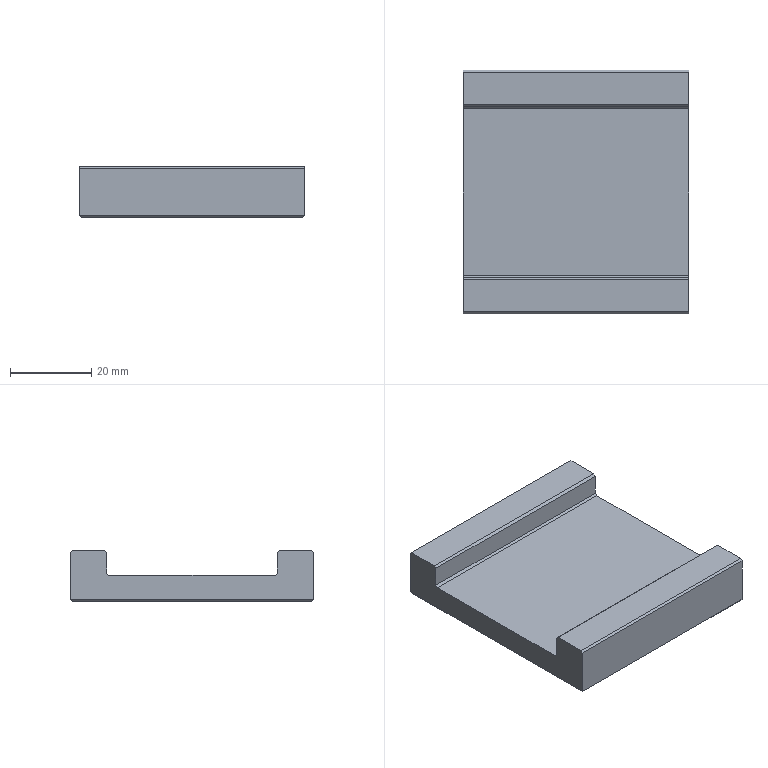Component | SolidWorks | SRS15WM-Slider-2-1 | 1 solid | 36 faces | box 55.5 x 60 x 12.6 mm | volume 27480 mm3 | plane 20 | cylinder 8 | cone 8 | commonest cylinder face diameters 3.3 x8
build123d program:
from build123d import *

# Parameters (mm, degrees)
BOSS_EXTRUDE1_DEPTH   = 55.5
CHAMFER1_SIZE         = 0.5
M4_TAPPED_HOLE1_D     = 3.3
M4_TAPPED_HOLE1_DEPTH = 6
M4_TAPPED_HOLE1_TIP   = 0.9914


with BuildPart() as part:
    # Sketch1 → Boss-Extrude1 (new body)
    with BuildSketch(Plane.XY):
        Polygon((9, 0), (9, 6.1), (51, 6.1), (51, 0), (60, 0), (60, 12.6), (0, 12.6), (0, 0), align=None)
    extrude(amount=BOSS_EXTRUDE1_DEPTH)

    # Chamfer1
    chamfer1_edges = [part.edges().sort_by_distance(p)[0] for p in [
        (0, 12.6, 27.75),
        (60, 12.6, 27.75),
        (60, 0, 27.75),
        (51, 0, 27.75),
        (51, 6.1, 27.75),
        (9, 6.1, 27.75),
        (9, 0, 27.75),
        (0, 0, 27.75),
        (30, 12.6, 55.5),
        (30, 12.6, 0),
    ]]
    chamfer(chamfer1_edges, length=CHAMFER1_SIZE)

    # M4 Tapped Hole1
    with Locations(Plane(origin=(0, 12.6, 0), x_dir=(1, 0, 0), z_dir=(0, 1, 0))):
        with Locations((7.5, -17.75), (52.5, -17.75), (52.5, -37.75), (7.5, -37.75)):
            Hole(M4_TAPPED_HOLE1_D / 2, depth=M4_TAPPED_HOLE1_DEPTH)
            with Locations((0, 0, -(M4_TAPPED_HOLE1_DEPTH + M4_TAPPED_HOLE1_TIP / 2))):  # 118° drill point
                Cone(0, M4_TAPPED_HOLE1_D / 2, M4_TAPPED_HOLE1_TIP, mode=Mode.SUBTRACT)


solid = part.part

# Placed as in the assembly
solid = solid.moved(Location((-73.445, 49.945, 33.151), (-90, 90, 0)))
STEP:
#1=COLOUR_RGB('',0.7922,0.8196,0.9333);
#2=FILL_AREA_STYLE_COLOUR('',#1);
#3=FILL_AREA_STYLE('',(#2));
#4=SURFACE_STYLE_FILL_AREA(#3);
#5=SURFACE_SIDE_STYLE('',(#4));
#6=SURFACE_STYLE_USAGE(.BOTH.,#5);
#7=PRESENTATION_STYLE_ASSIGNMENT((#6));
#8=CARTESIAN_POINT('',(-1.34,-0.1006,1.045));
#9=VERTEX_POINT('',#8);
#10=CARTESIAN_POINT('',(-1.47,-0.1006,1.045));
#11=VERTEX_POINT('',#10);
#12=CARTESIAN_POINT('',(-1.405,-0.1006,1.045));
#13=DIRECTION('',(-0.,0.,-1.));
#14=DIRECTION('',(-1.,0.,0.));
#15=AXIS2_PLACEMENT_3D('',#12,#13,#14);
#16=CIRCLE('',#15,0.06496);
#17=EDGE_CURVE('',#9,#11,#16,.T.);
#18=ORIENTED_EDGE('',*,*,#17,.F.);
#19=CARTESIAN_POINT('',(-1.34,-0.1006,0.8091));
#20=VERTEX_POINT('',#19);
#21=CARTESIAN_POINT('',(-1.34,-0.1006,0.8091));
#22=DIRECTION('',(-0.,0.,-1.));
#23=VECTOR('',#22,39.37);
#24=LINE('',#21,#23);
#25=EDGE_CURVE('',#9,#20,#24,.T.);
#26=ORIENTED_EDGE('',*,*,#25,.T.);
#27=CARTESIAN_POINT('',(-1.47,-0.1006,0.8091));
#28=VERTEX_POINT('',#27);
#29=CARTESIAN_POINT('',(-1.405,-0.1006,0.8091));
#30=DIRECTION('',(-0.,0.,-1.));
#31=DIRECTION('',(-1.,0.,0.));
#32=AXIS2_PLACEMENT_3D('',#29,#30,#31);
#33=CIRCLE('',#32,0.06496);
#34=EDGE_CURVE('',#20,#28,#33,.T.);
#35=ORIENTED_EDGE('',*,*,#34,.T.);
#36=CARTESIAN_POINT('',(-1.47,-0.1006,0.8091));
#37=DIRECTION('',(-0.,0.,-1.));
#38=VECTOR('',#37,39.37);
#39=LINE('',#36,#38);
#40=EDGE_CURVE('',#11,#28,#39,.T.);
#41=ORIENTED_EDGE('',*,*,#40,.F.);
#42=EDGE_LOOP('',(#18,#26,#35,#41));
#43=FACE_OUTER_BOUND('',#42,.T.);
#44=CARTESIAN_POINT('',(-1.405,-0.1006,0.8091));
#45=DIRECTION('',(-0.,0.,-1.));
#46=DIRECTION('',(-1.,0.,0.));
#47=AXIS2_PLACEMENT_3D('',#44,#45,#46);
#48=CYLINDRICAL_SURFACE('',#47,0.06496);
#49=ADVANCED_FACE('',(#43),#48,.F.);
#50=CARTESIAN_POINT('',(-1.405,-0.1006,1.084));
#51=VERTEX_POINT('',#50);
#52=CARTESIAN_POINT('',(-1.47,-0.1006,1.045));
#53=DIRECTION('',(-0.8572,0.,-0.515));
#54=VECTOR('',#53,39.37);
#55=LINE('',#52,#54);
#56=EDGE_CURVE('',#51,#11,#55,.T.);
#57=ORIENTED_EDGE('',*,*,#56,.F.);
#58=CARTESIAN_POINT('',(-1.34,-0.1006,1.045));
#59=DIRECTION('',(0.8572,-0.,-0.515));
#60=VECTOR('',#59,39.37);
#61=LINE('',#58,#60);
#62=EDGE_CURVE('',#51,#9,#61,.T.);
#63=ORIENTED_EDGE('',*,*,#62,.T.);
#64=ORIENTED_EDGE('',*,*,#17,.T.);
#65=EDGE_LOOP('',(#57,#63,#64));
#66=FACE_OUTER_BOUND('',#65,.T.);
#67=CARTESIAN_POINT('',(-1.405,-0.1006,1.045));
#68=DIRECTION('',(-0.,0.,-1.));
#69=DIRECTION('',(-1.,0.,0.));
#70=AXIS2_PLACEMENT_3D('',#67,#68,#69);
#71=CONICAL_SURFACE('',#70,0.06496,1.03);
#72=ADVANCED_FACE('',(#66),#71,.F.);
#73=CARTESIAN_POINT('',(-1.34,1.671,1.045));
#74=VERTEX_POINT('',#73);
#75=CARTESIAN_POINT('',(-1.47,1.671,1.045));
#76=VERTEX_POINT('',#75);
#77=CARTESIAN_POINT('',(-1.405,1.671,1.045));
#78=DIRECTION('',(-0.,0.,-1.));
#79=DIRECTION('',(-1.,0.,0.));
#80=AXIS2_PLACEMENT_3D('',#77,#78,#79);
#81=CIRCLE('',#80,0.06496);
#82=EDGE_CURVE('',#74,#76,#81,.T.);
#83=ORIENTED_EDGE('',*,*,#82,.F.);
#84=CARTESIAN_POINT('',(-1.34,1.671,0.8091));
#85=VERTEX_POINT('',#84);
#86=CARTESIAN_POINT('',(-1.34,1.671,0.8091));
#87=DIRECTION('',(-0.,0.,-1.));
#88=VECTOR('',#87,39.37);
#89=LINE('',#86,#88);
#90=EDGE_CURVE('',#74,#85,#89,.T.);
#91=ORIENTED_EDGE('',*,*,#90,.T.);
#92=CARTESIAN_POINT('',(-1.47,1.671,0.8091));
#93=VERTEX_POINT('',#92);
#94=CARTESIAN_POINT('',(-1.405,1.671,0.8091));
#95=DIRECTION('',(-0.,0.,-1.));
#96=DIRECTION('',(-1.,0.,0.));
#97=AXIS2_PLACEMENT_3D('',#94,#95,#96);
#98=CIRCLE('',#97,0.06496);
#99=EDGE_CURVE('',#85,#93,#98,.T.);
#100=ORIENTED_EDGE('',*,*,#99,.T.);
#101=CARTESIAN_POINT('',(-1.47,1.671,0.8091));
#102=DIRECTION('',(-0.,0.,-1.));
#103=VECTOR('',#102,39.37);
#104=LINE('',#101,#103);
#105=EDGE_CURVE('',#76,#93,#104,.T.);
#106=ORIENTED_EDGE('',*,*,#105,.F.);
#107=EDGE_LOOP('',(#83,#91,#100,#106));
#108=FACE_OUTER_BOUND('',#107,.T.);
#109=CARTESIAN_POINT('',(-1.405,1.671,0.8091));
#110=DIRECTION('',(-0.,0.,-1.));
#111=DIRECTION('',(-1.,0.,0.));
#112=AXIS2_PLACEMENT_3D('',#109,#110,#111);
#113=CYLINDRICAL_SURFACE('',#112,0.06496);
#114=ADVANCED_FACE('',(#108),#113,.F.);
#115=CARTESIAN_POINT('',(-1.405,1.671,1.084));
#116=VERTEX_POINT('',#115);
#117=CARTESIAN_POINT('',(-1.47,1.671,1.045));
#118=DIRECTION('',(-0.8572,0.,-0.515));
#119=VECTOR('',#118,39.37);
#120=LINE('',#117,#119);
#121=EDGE_CURVE('',#116,#76,#120,.T.);
#122=ORIENTED_EDGE('',*,*,#121,.F.);
#123=CARTESIAN_POINT('',(-1.34,1.671,1.045));
#124=DIRECTION('',(0.8572,-0.,-0.515));
#125=VECTOR('',#124,39.37);
#126=LINE('',#123,#125);
#127=EDGE_CURVE('',#116,#74,#126,.T.);
#128=ORIENTED_EDGE('',*,*,#127,.T.);
#129=ORIENTED_EDGE('',*,*,#82,.T.);
#130=EDGE_LOOP('',(#122,#128,#129));
#131=FACE_OUTER_BOUND('',#130,.T.);
#132=CARTESIAN_POINT('',(-1.405,1.671,1.045));
#133=DIRECTION('',(-0.,0.,-1.));
#134=DIRECTION('',(-1.,0.,0.));
#135=AXIS2_PLACEMENT_3D('',#132,#133,#134);
#136=CONICAL_SURFACE('',#135,0.06496,1.03);
#137=ADVANCED_FACE('',(#131),#136,.F.);
#138=CARTESIAN_POINT('',(-2.128,1.671,1.045));
#139=VERTEX_POINT('',#138);
#140=CARTESIAN_POINT('',(-2.258,1.671,1.045));
#141=VERTEX_POINT('',#140);
#142=CARTESIAN_POINT('',(-2.193,1.671,1.045));
#143=DIRECTION('',(-0.,0.,-1.));
#144=DIRECTION('',(-1.,0.,0.));
#145=AXIS2_PLACEMENT_3D('',#142,#143,#144);
#146=CIRCLE('',#145,0.06496);
#147=EDGE_CURVE('',#139,#141,#146,.T.);
#148=ORIENTED_EDGE('',*,*,#147,.F.);
#149=CARTESIAN_POINT('',(-2.128,1.671,0.8091));
#150=VERTEX_POINT('',#149);
#151=CARTESIAN_POINT('',(-2.128,1.671,0.8091));
#152=DIRECTION('',(-0.,0.,-1.));
#153=VECTOR('',#152,39.37);
#154=LINE('',#151,#153);
#155=EDGE_CURVE('',#139,#150,#154,.T.);
#156=ORIENTED_EDGE('',*,*,#155,.T.);
#157=CARTESIAN_POINT('',(-2.258,1.671,0.8091));
#158=VERTEX_POINT('',#157);
#159=CARTESIAN_POINT('',(-2.193,1.671,0.8091));
#160=DIRECTION('',(-0.,0.,-1.));
#161=DIRECTION('',(-1.,0.,0.));
#162=AXIS2_PLACEMENT_3D('',#159,#160,#161);
#163=CIRCLE('',#162,0.06496);
#164=EDGE_CURVE('',#150,#158,#163,.T.);
#165=ORIENTED_EDGE('',*,*,#164,.T.);
#166=CARTESIAN_POINT('',(-2.258,1.671,0.8091));
#167=DIRECTION('',(-0.,0.,-1.));
#168=VECTOR('',#167,39.37);
#169=LINE('',#166,#168);
#170=EDGE_CURVE('',#141,#158,#169,.T.);
#171=ORIENTED_EDGE('',*,*,#170,.F.);
#172=EDGE_LOOP('',(#148,#156,#165,#171));
#173=FACE_OUTER_BOUND('',#172,.T.);
#174=CARTESIAN_POINT('',(-2.193,1.671,0.8091));
#175=DIRECTION('',(-0.,0.,-1.));
#176=DIRECTION('',(-1.,0.,0.));
#177=AXIS2_PLACEMENT_3D('',#174,#175,#176);
#178=CYLINDRICAL_SURFACE('',#177,0.06496);
#179=ADVANCED_FACE('',(#173),#178,.F.);
#180=CARTESIAN_POINT('',(-2.193,1.671,1.084));
#181=VERTEX_POINT('',#180);
#182=CARTESIAN_POINT('',(-2.258,1.671,1.045));
#183=DIRECTION('',(-0.8572,0.,-0.515));
#184=VECTOR('',#183,39.37);
#185=LINE('',#182,#184);
#186=EDGE_CURVE('',#181,#141,#185,.T.);
#187=ORIENTED_EDGE('',*,*,#186,.F.);
#188=CARTESIAN_POINT('',(-2.128,1.671,1.045));
#189=DIRECTION('',(0.8572,-0.,-0.515));
#190=VECTOR('',#189,39.37);
#191=LINE('',#188,#190);
#192=EDGE_CURVE('',#181,#139,#191,.T.);
#193=ORIENTED_EDGE('',*,*,#192,.T.);
#194=ORIENTED_EDGE('',*,*,#147,.T.);
#195=EDGE_LOOP('',(#187,#193,#194));
#196=FACE_OUTER_BOUND('',#195,.T.);
#197=CARTESIAN_POINT('',(-2.193,1.671,1.045));
#198=DIRECTION('',(-0.,0.,-1.));
#199=DIRECTION('',(-1.,0.,0.));
#200=AXIS2_PLACEMENT_3D('',#197,#198,#199);
#201=CONICAL_SURFACE('',#200,0.06496,1.03);
#202=ADVANCED_FACE('',(#196),#201,.F.);
#203=CARTESIAN_POINT('',(-2.128,-0.1006,1.045));
#204=VERTEX_POINT('',#203);
#205=CARTESIAN_POINT('',(-2.258,-0.1006,1.045));
#206=VERTEX_POINT('',#205);
#207=CARTESIAN_POINT('',(-2.193,-0.1006,1.045));
#208=DIRECTION('',(-0.,0.,-1.));
#209=DIRECTION('',(-1.,0.,0.));
#210=AXIS2_PLACEMENT_3D('',#207,#208,#209);
#211=CIRCLE('',#210,0.06496);
#212=EDGE_CURVE('',#204,#206,#211,.T.);
#213=ORIENTED_EDGE('',*,*,#212,.F.);
#214=CARTESIAN_POINT('',(-2.128,-0.1006,0.8091));
#215=VERTEX_POINT('',#214);
#216=CARTESIAN_POINT('',(-2.128,-0.1006,0.8091));
#217=DIRECTION('',(-0.,0.,-1.));
#218=VECTOR('',#217,39.37);
#219=LINE('',#216,#218);
#220=EDGE_CURVE('',#204,#215,#219,.T.);
#221=ORIENTED_EDGE('',*,*,#220,.T.);
#222=CARTESIAN_POINT('',(-2.258,-0.1006,0.8091));
#223=VERTEX_POINT('',#222);
#224=CARTESIAN_POINT('',(-2.193,-0.1006,0.8091));
#225=DIRECTION('',(-0.,0.,-1.));
#226=DIRECTION('',(-1.,0.,0.));
#227=AXIS2_PLACEMENT_3D('',#224,#225,#226);
#228=CIRCLE('',#227,0.06496);
#229=EDGE_CURVE('',#215,#223,#228,.T.);
#230=ORIENTED_EDGE('',*,*,#229,.T.);
#231=CARTESIAN_POINT('',(-2.258,-0.1006,0.8091));
#232=DIRECTION('',(-0.,0.,-1.));
#233=VECTOR('',#232,39.37);
#234=LINE('',#231,#233);
#235=EDGE_CURVE('',#206,#223,#234,.T.);
#236=ORIENTED_EDGE('',*,*,#235,.F.);
#237=EDGE_LOOP('',(#213,#221,#230,#236));
#238=FACE_OUTER_BOUND('',#237,.T.);
#239=CARTESIAN_POINT('',(-2.193,-0.1006,0.8091));
#240=DIRECTION('',(-0.,0.,-1.));
#241=DIRECTION('',(-1.,0.,0.));
#242=AXIS2_PLACEMENT_3D('',#239,#240,#241);
#243=CYLINDRICAL_SURFACE('',#242,0.06496);
#244=ADVANCED_FACE('',(#238),#243,.F.);
#245=CARTESIAN_POINT('',(-2.193,-0.1006,1.084));
#246=VERTEX_POINT('',#245);
#247=CARTESIAN_POINT('',(-2.258,-0.1006,1.045));
#248=DIRECTION('',(-0.8572,0.,-0.515));
#249=VECTOR('',#248,39.37);
#250=LINE('',#247,#249);
#251=EDGE_CURVE('',#246,#206,#250,.T.);
#252=ORIENTED_EDGE('',*,*,#251,.F.);
#253=CARTESIAN_POINT('',(-2.128,-0.1006,1.045));
#254=DIRECTION('',(0.8572,-0.,-0.515));
#255=VECTOR('',#254,39.37);
#256=LINE('',#253,#255);
#257=EDGE_CURVE('',#246,#204,#256,.T.);
#258=ORIENTED_EDGE('',*,*,#257,.T.);
#259=ORIENTED_EDGE('',*,*,#212,.T.);
#260=EDGE_LOOP('',(#252,#258,#259));
#261=FACE_OUTER_BOUND('',#260,.T.);
#262=CARTESIAN_POINT('',(-2.193,-0.1006,1.045));
#263=DIRECTION('',(-0.,0.,-1.));
#264=DIRECTION('',(-1.,0.,0.));
#265=AXIS2_PLACEMENT_3D('',#262,#263,#264);
#266=CONICAL_SURFACE('',#265,0.06496,1.03);
#267=ADVANCED_FACE('',(#261),#266,.F.);
#268=CARTESIAN_POINT('',(-2.892,-0.3959,0.8288));
#269=VERTEX_POINT('',#268);
#270=CARTESIAN_POINT('',(-2.892,-0.3959,1.285));
#271=VERTEX_POINT('',#270);
#272=CARTESIAN_POINT('',(-2.892,-0.3959,1.305));
#273=DIRECTION('',(0.,-0.,1.));
#274=VECTOR('',#273,39.37);
#275=LINE('',#272,#274);
#276=EDGE_CURVE('',#269,#271,#275,.T.);
#277=ORIENTED_EDGE('',*,*,#276,.F.);
#278=CARTESIAN_POINT('',(-0.7065,-0.3959,0.8288));
#279=VERTEX_POINT('',#278);
#280=CARTESIAN_POINT('',(-2.892,-0.3959,0.8288));
#281=DIRECTION('',(1.,-0.,-0.));
#282=VECTOR('',#281,39.37);
#283=LINE('',#280,#282);
#284=EDGE_CURVE('',#269,#279,#283,.T.);
#285=ORIENTED_EDGE('',*,*,#284,.T.);
#286=CARTESIAN_POINT('',(-0.7065,-0.3959,1.285));
#287=VERTEX_POINT('',#286);
#288=CARTESIAN_POINT('',(-0.7065,-0.3959,1.305));
#289=DIRECTION('',(0.,-0.,1.));
#290=VECTOR('',#289,39.37);
#291=LINE('',#288,#290);
#292=EDGE_CURVE('',#279,#287,#291,.T.);
#293=ORIENTED_EDGE('',*,*,#292,.T.);
#294=CARTESIAN_POINT('',(-2.892,-0.3959,1.285));
#295=DIRECTION('',(-1.,0.,0.));
#296=VECTOR('',#295,39.37);
#297=LINE('',#294,#296);
#298=EDGE_CURVE('',#287,#271,#297,.T.);
#299=ORIENTED_EDGE('',*,*,#298,.T.);
#300=EDGE_LOOP('',(#277,#285,#293,#299));
#301=FACE_OUTER_BOUND('',#300,.T.);
#302=CARTESIAN_POINT('',(-2.892,-0.3959,1.305));
#303=DIRECTION('',(0.,1.,0.));
#304=DIRECTION('',(1.,-0.,-0.));
#305=AXIS2_PLACEMENT_3D('',#302,#303,#304);
#306=PLANE('',#305);
#307=ADVANCED_FACE('',(#301),#306,.F.);
#308=CARTESIAN_POINT('',(-0.7065,-0.3762,1.305));
#309=VERTEX_POINT('',#308);
#310=CARTESIAN_POINT('',(-0.7065,-0.0612,1.305));
#311=VERTEX_POINT('',#310);
#312=CARTESIAN_POINT('',(-0.7065,-0.3959,1.305));
#313=DIRECTION('',(0.,1.,0.));
#314=VECTOR('',#313,39.37);
#315=LINE('',#312,#314);
#316=EDGE_CURVE('',#309,#311,#315,.T.);
#317=ORIENTED_EDGE('',*,*,#316,.T.);
#318=CARTESIAN_POINT('',(-2.892,-0.0612,1.305));
#319=VERTEX_POINT('',#318);
#320=CARTESIAN_POINT('',(-2.892,-0.0612,1.305));
#321=DIRECTION('',(-1.,0.,0.));
#322=VECTOR('',#321,39.37);
#323=LINE('',#320,#322);
#324=EDGE_CURVE('',#311,#319,#323,.T.);
#325=ORIENTED_EDGE('',*,*,#324,.T.);
#326=CARTESIAN_POINT('',(-2.892,-0.3762,1.305));
#327=VERTEX_POINT('',#326);
#328=CARTESIAN_POINT('',(-2.892,-0.3959,1.305));
#329=DIRECTION('',(0.,1.,0.));
#330=VECTOR('',#329,39.37);
#331=LINE('',#328,#330);
#332=EDGE_CURVE('',#327,#319,#331,.T.);
#333=ORIENTED_EDGE('',*,*,#332,.F.);
#334=CARTESIAN_POINT('',(-2.892,-0.3762,1.305));
#335=DIRECTION('',(1.,-0.,-0.));
#336=VECTOR('',#335,39.37);
#337=LINE('',#334,#336);
#338=EDGE_CURVE('',#327,#309,#337,.T.);
#339=ORIENTED_EDGE('',*,*,#338,.T.);
#340=EDGE_LOOP('',(#317,#325,#333,#339));
#341=FACE_OUTER_BOUND('',#340,.T.);
#342=CARTESIAN_POINT('',(-2.892,-0.3959,1.305));
#343=DIRECTION('',(-0.,0.,-1.));
#344=DIRECTION('',(-1.,0.,0.));
#345=AXIS2_PLACEMENT_3D('',#342,#343,#344);
#346=PLANE('',#345);
#347=ADVANCED_FACE('',(#341),#346,.F.);
#348=CARTESIAN_POINT('',(-0.7065,-0.04152,1.285));
#349=VERTEX_POINT('',#348);
#350=CARTESIAN_POINT('',(-0.7065,-0.04152,1.085));
#351=VERTEX_POINT('',#350);
#352=CARTESIAN_POINT('',(-0.7065,-0.04152,1.305));
#353=DIRECTION('',(-0.,0.,-1.));
#354=VECTOR('',#353,39.37);
#355=LINE('',#352,#354);
#356=EDGE_CURVE('',#349,#351,#355,.T.);
#357=ORIENTED_EDGE('',*,*,#356,.T.);
#358=CARTESIAN_POINT('',(-2.892,-0.04152,1.085));
#359=VERTEX_POINT('',#358);
#360=CARTESIAN_POINT('',(-2.892,-0.04152,1.085));
#361=DIRECTION('',(-1.,0.,0.));
#362=VECTOR('',#361,39.37);
#363=LINE('',#360,#362);
#364=EDGE_CURVE('',#351,#359,#363,.T.);
#365=ORIENTED_EDGE('',*,*,#364,.T.);
#366=CARTESIAN_POINT('',(-2.892,-0.04152,1.285));
#367=VERTEX_POINT('',#366);
#368=CARTESIAN_POINT('',(-2.892,-0.04152,1.305));
#369=DIRECTION('',(-0.,0.,-1.));
#370=VECTOR('',#369,39.37);
#371=LINE('',#368,#370);
#372=EDGE_CURVE('',#367,#359,#371,.T.);
#373=ORIENTED_EDGE('',*,*,#372,.F.);
#374=CARTESIAN_POINT('',(-2.892,-0.04152,1.285));
#375=DIRECTION('',(1.,-0.,-0.));
#376=VECTOR('',#375,39.37);
#377=LINE('',#374,#376);
#378=EDGE_CURVE('',#367,#349,#377,.T.);
#379=ORIENTED_EDGE('',*,*,#378,.T.);
#380=EDGE_LOOP('',(#357,#365,#373,#379));
#381=FACE_OUTER_BOUND('',#380,.T.);
#382=CARTESIAN_POINT('',(-2.892,-0.04152,1.305));
#383=DIRECTION('',(-0.,-1.,-0.));
#384=DIRECTION('',(-1.,0.,0.));
#385=AXIS2_PLACEMENT_3D('',#382,#383,#384);
#386=PLANE('',#385);
#387=ADVANCED_FACE('',(#381),#386,.F.);
#388=CARTESIAN_POINT('',(-0.7065,-0.02183,1.065));
#389=VERTEX_POINT('',#388);
#390=CARTESIAN_POINT('',(-0.7065,1.592,1.065));
#391=VERTEX_POINT('',#390);
#392=CARTESIAN_POINT('',(-0.7065,-0.04152,1.065));
#393=DIRECTION('',(0.,1.,0.));
#394=VECTOR('',#393,39.37);
#395=LINE('',#392,#394);
#396=EDGE_CURVE('',#389,#391,#395,.T.);
#397=ORIENTED_EDGE('',*,*,#396,.T.);
#398=CARTESIAN_POINT('',(-2.892,1.592,1.065));
#399=VERTEX_POINT('',#398);
#400=CARTESIAN_POINT('',(-2.892,1.592,1.065));
#401=DIRECTION('',(-1.,0.,0.));
#402=VECTOR('',#401,39.37);
#403=LINE('',#400,#402);
#404=EDGE_CURVE('',#391,#399,#403,.T.);
#405=ORIENTED_EDGE('',*,*,#404,.T.);
#406=CARTESIAN_POINT('',(-2.892,-0.02183,1.065));
#407=VERTEX_POINT('',#406);
#408=CARTESIAN_POINT('',(-2.892,-0.04152,1.065));
#409=DIRECTION('',(0.,1.,0.));
#410=VECTOR('',#409,39.37);
#411=LINE('',#408,#410);
#412=EDGE_CURVE('',#407,#399,#411,.T.);
#413=ORIENTED_EDGE('',*,*,#412,.F.);
#414=CARTESIAN_POINT('',(-0.7065,-0.02183,1.065));
#415=DIRECTION('',(1.,-0.,-0.));
#416=VECTOR('',#415,39.37);
#417=LINE('',#414,#416);
#418=EDGE_CURVE('',#407,#389,#417,.T.);
#419=ORIENTED_EDGE('',*,*,#418,.T.);
#420=EDGE_LOOP('',(#397,#405,#413,#419));
#421=FACE_OUTER_BOUND('',#420,.T.);
#422=CARTESIAN_POINT('',(-2.892,-0.04152,1.065));
#423=DIRECTION('',(-0.,0.,-1.));
#424=DIRECTION('',(-1.,0.,0.));
#425=AXIS2_PLACEMENT_3D('',#422,#423,#424);
#426=PLANE('',#425);
#427=ADVANCED_FACE('',(#421),#426,.F.);
#428=CARTESIAN_POINT('',(-0.7065,1.612,1.085));
#429=VERTEX_POINT('',#428);
#430=CARTESIAN_POINT('',(-0.7065,1.612,1.285));
#431=VERTEX_POINT('',#430);
#432=CARTESIAN_POINT('',(-0.7065,1.612,1.065));
#433=DIRECTION('',(0.,-0.,1.));
#434=VECTOR('',#433,39.37);
#435=LINE('',#432,#434);
#436=EDGE_CURVE('',#429,#431,#435,.T.);
#437=ORIENTED_EDGE('',*,*,#436,.T.);
#438=CARTESIAN_POINT('',(-2.892,1.612,1.285));
#439=VERTEX_POINT('',#438);
#440=CARTESIAN_POINT('',(-2.892,1.612,1.285));
#441=DIRECTION('',(-1.,0.,0.));
#442=VECTOR('',#441,39.37);
#443=LINE('',#440,#442);
#444=EDGE_CURVE('',#431,#439,#443,.T.);
#445=ORIENTED_EDGE('',*,*,#444,.T.);
#446=CARTESIAN_POINT('',(-2.892,1.612,1.085));
#447=VERTEX_POINT('',#446);
#448=CARTESIAN_POINT('',(-2.892,1.612,1.065));
#449=DIRECTION('',(0.,-0.,1.));
#450=VECTOR('',#449,39.37);
#451=LINE('',#448,#450);
#452=EDGE_CURVE('',#447,#439,#451,.T.);
#453=ORIENTED_EDGE('',*,*,#452,.F.);
#454=CARTESIAN_POINT('',(-0.7065,1.612,1.085));
#455=DIRECTION('',(1.,-0.,-0.));
#456=VECTOR('',#455,39.37);
#457=LINE('',#454,#456);
#458=EDGE_CURVE('',#447,#429,#457,.T.);
#459=ORIENTED_EDGE('',*,*,#458,.T.);
#460=EDGE_LOOP('',(#437,#445,#453,#459));
#461=FACE_OUTER_BOUND('',#460,.T.);
#462=CARTESIAN_POINT('',(-2.892,1.612,1.065));
#463=DIRECTION('',(0.,1.,0.));
#464=DIRECTION('',(1.,-0.,-0.));
#465=AXIS2_PLACEMENT_3D('',#462,#463,#464);
#466=PLANE('',#465);
#467=ADVANCED_FACE('',(#461),#466,.F.);
#468=CARTESIAN_POINT('',(-2.892,1.632,1.305));
#469=VERTEX_POINT('',#468);
#470=CARTESIAN_POINT('',(-2.892,1.947,1.305));
#471=VERTEX_POINT('',#470);
#472=CARTESIAN_POINT('',(-2.892,1.612,1.305));
#473=DIRECTION('',(0.,1.,0.));
#474=VECTOR('',#473,39.37);
#475=LINE('',#472,#474);
#476=EDGE_CURVE('',#469,#471,#475,.T.);
#477=ORIENTED_EDGE('',*,*,#476,.F.);
#478=CARTESIAN_POINT('',(-0.7065,1.632,1.305));
#479=VERTEX_POINT('',#478);
#480=CARTESIAN_POINT('',(-2.892,1.632,1.305));
#481=DIRECTION('',(1.,-0.,-0.));
#482=VECTOR('',#481,39.37);
#483=LINE('',#480,#482);
#484=EDGE_CURVE('',#469,#479,#483,.T.);
#485=ORIENTED_EDGE('',*,*,#484,.T.);
#486=CARTESIAN_POINT('',(-0.7065,1.947,1.305));
#487=VERTEX_POINT('',#486);
#488=CARTESIAN_POINT('',(-0.7065,1.612,1.305));
#489=DIRECTION('',(0.,1.,0.));
#490=VECTOR('',#489,39.37);
#491=LINE('',#488,#490);
#492=EDGE_CURVE('',#479,#487,#491,.T.);
#493=ORIENTED_EDGE('',*,*,#492,.T.);
#494=CARTESIAN_POINT('',(-2.892,1.947,1.305));
#495=DIRECTION('',(-1.,0.,0.));
#496=VECTOR('',#495,39.37);
#497=LINE('',#494,#496);
#498=EDGE_CURVE('',#487,#471,#497,.T.);
#499=ORIENTED_EDGE('',*,*,#498,.T.);
#500=EDGE_LOOP('',(#477,#485,#493,#499));
#501=FACE_OUTER_BOUND('',#500,.T.);
#502=CARTESIAN_POINT('',(-2.892,1.612,1.305));
#503=DIRECTION('',(-0.,0.,-1.));
#504=DIRECTION('',(-1.,0.,0.));
#505=AXIS2_PLACEMENT_3D('',#502,#503,#504);
#506=PLANE('',#505);
#507=ADVANCED_FACE('',(#501),#506,.F.);
#508=CARTESIAN_POINT('',(-0.7065,1.966,1.285));
#509=VERTEX_POINT('',#508);
#510=CARTESIAN_POINT('',(-0.7065,1.966,0.8288));
#511=VERTEX_POINT('',#510);
#512=CARTESIAN_POINT('',(-0.7065,1.966,1.305));
#513=DIRECTION('',(-0.,0.,-1.));
#514=VECTOR('',#513,39.37);
#515=LINE('',#512,#514);
#516=EDGE_CURVE('',#509,#511,#515,.T.);
#517=ORIENTED_EDGE('',*,*,#516,.T.);
#518=CARTESIAN_POINT('',(-2.892,1.966,0.8288));
#519=VERTEX_POINT('',#518);
#520=CARTESIAN_POINT('',(-2.892,1.966,0.8288));
#521=DIRECTION('',(-1.,0.,0.));
#522=VECTOR('',#521,39.37);
#523=LINE('',#520,#522);
#524=EDGE_CURVE('',#511,#519,#523,.T.);
#525=ORIENTED_EDGE('',*,*,#524,.T.);
#526=CARTESIAN_POINT('',(-2.892,1.966,1.285));
#527=VERTEX_POINT('',#526);
#528=CARTESIAN_POINT('',(-2.892,1.966,1.305));
#529=DIRECTION('',(-0.,0.,-1.));
#530=VECTOR('',#529,39.37);
#531=LINE('',#528,#530);
#532=EDGE_CURVE('',#527,#519,#531,.T.);
#533=ORIENTED_EDGE('',*,*,#532,.F.);
#534=CARTESIAN_POINT('',(-2.892,1.966,1.285));
#535=DIRECTION('',(1.,-0.,-0.));
#536=VECTOR('',#535,39.37);
#537=LINE('',#534,#536);
#538=EDGE_CURVE('',#527,#509,#537,.T.);
#539=ORIENTED_EDGE('',*,*,#538,.T.);
#540=EDGE_LOOP('',(#517,#525,#533,#539));
#541=FACE_OUTER_BOUND('',#540,.T.);
#542=CARTESIAN_POINT('',(-2.892,1.966,1.305));
#543=DIRECTION('',(-0.,-1.,-0.));
#544=DIRECTION('',(-1.,0.,0.));
#545=AXIS2_PLACEMENT_3D('',#542,#543,#544);
#546=PLANE('',#545);
#547=ADVANCED_FACE('',(#541),#546,.F.);
#548=CARTESIAN_POINT('',(-1.405,-0.1006,0.8091));
#549=DIRECTION('',(-0.,0.,-1.));
#550=DIRECTION('',(-1.,0.,0.));
#551=AXIS2_PLACEMENT_3D('',#548,#549,#550);
#552=CIRCLE('',#551,0.06496);
#553=EDGE_CURVE('',#28,#20,#552,.T.);
#554=ORIENTED_EDGE('',*,*,#553,.F.);
#555=ORIENTED_EDGE('',*,*,#34,.F.);
#556=EDGE_LOOP('',(#554,#555));
#557=FACE_BOUND('',#556,.T.);
#558=CARTESIAN_POINT('',(-1.405,1.671,0.8091));
#559=DIRECTION('',(-0.,0.,-1.));
#560=DIRECTION('',(-1.,0.,0.));
#561=AXIS2_PLACEMENT_3D('',#558,#559,#560);
#562=CIRCLE('',#561,0.06496);
#563=EDGE_CURVE('',#93,#85,#562,.T.);
#564=ORIENTED_EDGE('',*,*,#563,.F.);
#565=ORIENTED_EDGE('',*,*,#99,.F.);
#566=EDGE_LOOP('',(#564,#565));
#567=FACE_BOUND('',#566,.T.);
#568=CARTESIAN_POINT('',(-2.193,1.671,0.8091));
#569=DIRECTION('',(-0.,0.,-1.));
#570=DIRECTION('',(-1.,0.,0.));
#571=AXIS2_PLACEMENT_3D('',#568,#569,#570);
#572=CIRCLE('',#571,0.06496);
#573=EDGE_CURVE('',#158,#150,#572,.T.);
#574=ORIENTED_EDGE('',*,*,#573,.F.);
#575=ORIENTED_EDGE('',*,*,#164,.F.);
#576=EDGE_LOOP('',(#574,#575));
#577=FACE_BOUND('',#576,.T.);
#578=CARTESIAN_POINT('',(-2.193,-0.1006,0.8091));
#579=DIRECTION('',(-0.,0.,-1.));
#580=DIRECTION('',(-1.,0.,0.));
#581=AXIS2_PLACEMENT_3D('',#578,#579,#580);
#582=CIRCLE('',#581,0.06496);
#583=EDGE_CURVE('',#223,#215,#582,.T.);
#584=ORIENTED_EDGE('',*,*,#583,.F.);
#585=ORIENTED_EDGE('',*,*,#229,.F.);
#586=EDGE_LOOP('',(#584,#585));
#587=FACE_BOUND('',#586,.T.);
#588=CARTESIAN_POINT('',(-2.872,-0.3762,0.8091));
#589=VERTEX_POINT('',#588);
#590=CARTESIAN_POINT('',(-2.872,1.947,0.8091));
#591=VERTEX_POINT('',#590);
#592=CARTESIAN_POINT('',(-2.872,-0.3959,0.8091));
#593=DIRECTION('',(0.,1.,0.));
#594=VECTOR('',#593,39.37);
#595=LINE('',#592,#594);
#596=EDGE_CURVE('',#589,#591,#595,.T.);
#597=ORIENTED_EDGE('',*,*,#596,.T.);
#598=CARTESIAN_POINT('',(-0.7262,1.947,0.8091));
#599=VERTEX_POINT('',#598);
#600=CARTESIAN_POINT('',(-2.892,1.947,0.8091));
#601=DIRECTION('',(1.,-0.,-0.));
#602=VECTOR('',#601,39.37);
#603=LINE('',#600,#602);
#604=EDGE_CURVE('',#591,#599,#603,.T.);
#605=ORIENTED_EDGE('',*,*,#604,.T.);
#606=CARTESIAN_POINT('',(-0.7262,-0.3762,0.8091));
#607=VERTEX_POINT('',#606);
#608=CARTESIAN_POINT('',(-0.7262,-0.3959,0.8091));
#609=DIRECTION('',(-0.,-1.,-0.));
#610=VECTOR('',#609,39.37);
#611=LINE('',#608,#610);
#612=EDGE_CURVE('',#599,#607,#611,.T.);
#613=ORIENTED_EDGE('',*,*,#612,.T.);
#614=CARTESIAN_POINT('',(-2.892,-0.3762,0.8091));
#615=DIRECTION('',(-1.,0.,0.));
#616=VECTOR('',#615,39.37);
#617=LINE('',#614,#616);
#618=EDGE_CURVE('',#607,#589,#617,.T.);
#619=ORIENTED_EDGE('',*,*,#618,.T.);
#620=EDGE_LOOP('',(#597,#605,#613,#619));
#621=FACE_OUTER_BOUND('',#620,.T.);
#622=CARTESIAN_POINT('',(-2.892,-0.3959,0.8091));
#623=DIRECTION('',(0.,-0.,1.));
#624=DIRECTION('',(1.,-0.,-0.));
#625=AXIS2_PLACEMENT_3D('',#622,#623,#624);
#626=PLANE('',#625);
#627=ADVANCED_FACE('',(#557,#567,#577,#587,#621),#626,.F.);
#628=ORIENTED_EDGE('',*,*,#532,.T.);
#629=CARTESIAN_POINT('',(-2.892,-0.3959,0.8288));
#630=DIRECTION('',(-0.,-1.,-0.));
#631=VECTOR('',#630,39.37);
#632=LINE('',#629,#631);
#633=EDGE_CURVE('',#519,#269,#632,.T.);
#634=ORIENTED_EDGE('',*,*,#633,.T.);
#635=ORIENTED_EDGE('',*,*,#276,.T.);
#636=CARTESIAN_POINT('',(-2.892,-0.3762,1.305));
#637=DIRECTION('',(0.,0.7071,0.7071));
#638=VECTOR('',#637,39.37);
#639=LINE('',#636,#638);
#640=EDGE_CURVE('',#271,#327,#639,.T.);
#641=ORIENTED_EDGE('',*,*,#640,.T.);
#642=ORIENTED_EDGE('',*,*,#332,.T.);
#643=CARTESIAN_POINT('',(-2.892,-0.04152,1.285));
#644=DIRECTION('',(0.,0.7071,-0.7071));
#645=VECTOR('',#644,39.37);
#646=LINE('',#643,#645);
#647=EDGE_CURVE('',#319,#367,#646,.T.);
#648=ORIENTED_EDGE('',*,*,#647,.T.);
#649=ORIENTED_EDGE('',*,*,#372,.T.);
#650=CARTESIAN_POINT('',(-2.892,-0.3289,1.372));
#651=DIRECTION('',(0.,0.7071,-0.7071));
#652=VECTOR('',#651,39.37);
#653=LINE('',#650,#652);
#654=EDGE_CURVE('',#359,#407,#653,.T.);
#655=ORIENTED_EDGE('',*,*,#654,.T.);
#656=ORIENTED_EDGE('',*,*,#412,.T.);
#657=CARTESIAN_POINT('',(-2.892,0.7183,0.191));
#658=DIRECTION('',(0.,0.7071,0.7071));
#659=VECTOR('',#658,39.37);
#660=LINE('',#657,#659);
#661=EDGE_CURVE('',#399,#447,#660,.T.);
#662=ORIENTED_EDGE('',*,*,#661,.T.);
#663=ORIENTED_EDGE('',*,*,#452,.T.);
#664=CARTESIAN_POINT('',(-2.892,1.632,1.305));
#665=DIRECTION('',(0.,0.7071,0.7071));
#666=VECTOR('',#665,39.37);
#667=LINE('',#664,#666);
#668=EDGE_CURVE('',#439,#469,#667,.T.);
#669=ORIENTED_EDGE('',*,*,#668,.T.);
#670=ORIENTED_EDGE('',*,*,#476,.T.);
#671=CARTESIAN_POINT('',(-2.892,1.966,1.285));
#672=DIRECTION('',(0.,0.7071,-0.7071));
#673=VECTOR('',#672,39.37);
#674=LINE('',#671,#673);
#675=EDGE_CURVE('',#471,#527,#674,.T.);
#676=ORIENTED_EDGE('',*,*,#675,.T.);
#677=EDGE_LOOP('',(#628,#634,#635,#641,#642,#648,#649,#655,#656,#662,#663,#669,#670,#676));
#678=FACE_OUTER_BOUND('',#677,.T.);
#679=CARTESIAN_POINT('',(-2.892,-0.3959,1.305));
#680=DIRECTION('',(1.,-0.,-0.));
#681=DIRECTION('',(-0.,-1.,-0.));
#682=AXIS2_PLACEMENT_3D('',#679,#680,#681);
#683=PLANE('',#682);
#684=ADVANCED_FACE('',(#678),#683,.F.);
#685=ORIENTED_EDGE('',*,*,#292,.F.);
#686=CARTESIAN_POINT('',(-0.7065,1.966,0.8288));
#687=DIRECTION('',(0.,1.,0.));
#688=VECTOR('',#687,39.37);
#689=LINE('',#686,#688);
#690=EDGE_CURVE('',#279,#511,#689,.T.);
#691=ORIENTED_EDGE('',*,*,#690,.T.);
#692=ORIENTED_EDGE('',*,*,#516,.F.);
#693=CARTESIAN_POINT('',(-0.7065,0.7754,2.476));
#694=DIRECTION('',(-0.,-0.7071,0.7071));
#695=VECTOR('',#694,39.37);
#696=LINE('',#693,#695);
#697=EDGE_CURVE('',#509,#487,#696,.T.);
#698=ORIENTED_EDGE('',*,*,#697,.T.);
#699=ORIENTED_EDGE('',*,*,#492,.F.);
#700=CARTESIAN_POINT('',(-0.7065,0.6179,0.2914));
#701=DIRECTION('',(-0.,-0.7071,-0.7071));
#702=VECTOR('',#701,39.37);
#703=LINE('',#700,#702);
#704=EDGE_CURVE('',#479,#431,#703,.T.);
#705=ORIENTED_EDGE('',*,*,#704,.T.);
#706=ORIENTED_EDGE('',*,*,#436,.F.);
#707=CARTESIAN_POINT('',(-0.7065,1.612,1.085));
#708=DIRECTION('',(-0.,-0.7071,-0.7071));
#709=VECTOR('',#708,39.37);
#710=LINE('',#707,#709);
#711=EDGE_CURVE('',#429,#391,#710,.T.);
#712=ORIENTED_EDGE('',*,*,#711,.T.);
#713=ORIENTED_EDGE('',*,*,#396,.F.);
#714=CARTESIAN_POINT('',(-0.7065,-0.02183,1.065));
#715=DIRECTION('',(-0.,-0.7071,0.7071));
#716=VECTOR('',#715,39.37);
#717=LINE('',#714,#716);
#718=EDGE_CURVE('',#389,#351,#717,.T.);
#719=ORIENTED_EDGE('',*,*,#718,.T.);
#720=ORIENTED_EDGE('',*,*,#356,.F.);
#721=CARTESIAN_POINT('',(-0.7065,-0.2285,1.472));
#722=DIRECTION('',(-0.,-0.7071,0.7071));
#723=VECTOR('',#722,39.37);
#724=LINE('',#721,#723);
#725=EDGE_CURVE('',#349,#311,#724,.T.);
#726=ORIENTED_EDGE('',*,*,#725,.T.);
#727=ORIENTED_EDGE('',*,*,#316,.F.);
#728=CARTESIAN_POINT('',(-0.7065,-0.386,1.295));
#729=DIRECTION('',(-0.,-0.7071,-0.7071));
#730=VECTOR('',#729,39.37);
#731=LINE('',#728,#730);
#732=EDGE_CURVE('',#309,#287,#731,.T.);
#733=ORIENTED_EDGE('',*,*,#732,.T.);
#734=EDGE_LOOP('',(#685,#691,#692,#698,#699,#705,#706,#712,#713,#719,#720,#726,#727,#733));
#735=FACE_OUTER_BOUND('',#734,.T.);
#736=CARTESIAN_POINT('',(-0.7065,-0.3959,1.305));
#737=DIRECTION('',(1.,-0.,-0.));
#738=DIRECTION('',(-0.,-1.,-0.));
#739=AXIS2_PLACEMENT_3D('',#736,#737,#738);
#740=PLANE('',#739);
#741=ADVANCED_FACE('',(#735),#740,.T.);
#742=CARTESIAN_POINT('',(-0.7196,-0.3827,0.8156));
#743=DIRECTION('',(-0.5774,0.5774,-0.5774));
#744=VECTOR('',#743,39.37);
#745=LINE('',#742,#744);
#746=EDGE_CURVE('',#279,#607,#745,.T.);
#747=ORIENTED_EDGE('',*,*,#746,.F.);
#748=ORIENTED_EDGE('',*,*,#284,.F.);
#749=CARTESIAN_POINT('',(-2.892,-0.3959,0.8288));
#750=DIRECTION('',(-0.5774,-0.5774,0.5774));
#751=VECTOR('',#750,39.37);
#752=LINE('',#749,#751);
#753=EDGE_CURVE('',#589,#269,#752,.T.);
#754=ORIENTED_EDGE('',*,*,#753,.F.);
#755=ORIENTED_EDGE('',*,*,#618,.F.);
#756=EDGE_LOOP('',(#747,#748,#754,#755));
#757=FACE_OUTER_BOUND('',#756,.T.);
#758=CARTESIAN_POINT('',(-2.892,-0.3959,0.8288));
#759=DIRECTION('',(0.,0.7071,0.7071));
#760=DIRECTION('',(1.,-0.,-0.));
#761=AXIS2_PLACEMENT_3D('',#758,#759,#760);
#762=PLANE('',#761);
#763=ADVANCED_FACE('',(#757),#762,.F.);
#764=ORIENTED_EDGE('',*,*,#753,.T.);
#765=ORIENTED_EDGE('',*,*,#633,.F.);
#766=CARTESIAN_POINT('',(-2.104,1.179,0.04137));
#767=DIRECTION('',(-0.5774,0.5774,0.5774));
#768=VECTOR('',#767,39.37);
#769=LINE('',#766,#768);
#770=EDGE_CURVE('',#591,#519,#769,.T.);
#771=ORIENTED_EDGE('',*,*,#770,.F.);
#772=ORIENTED_EDGE('',*,*,#596,.F.);
#773=EDGE_LOOP('',(#764,#765,#771,#772));
#774=FACE_OUTER_BOUND('',#773,.T.);
#775=CARTESIAN_POINT('',(-2.892,-0.3959,0.8288));
#776=DIRECTION('',(0.7071,-0.,0.7071));
#777=DIRECTION('',(-0.,-1.,-0.));
#778=AXIS2_PLACEMENT_3D('',#775,#776,#777);
#779=PLANE('',#778);
#780=ADVANCED_FACE('',(#774),#779,.F.);
#781=ORIENTED_EDGE('',*,*,#746,.T.);
#782=ORIENTED_EDGE('',*,*,#612,.F.);
#783=CARTESIAN_POINT('',(-1.507,1.166,0.02824));
#784=DIRECTION('',(-0.5774,-0.5774,-0.5774));
#785=VECTOR('',#784,39.37);
#786=LINE('',#783,#785);
#787=EDGE_CURVE('',#511,#599,#786,.T.);
#788=ORIENTED_EDGE('',*,*,#787,.F.);
#789=ORIENTED_EDGE('',*,*,#690,.F.);
#790=EDGE_LOOP('',(#781,#782,#788,#789));
#791=FACE_OUTER_BOUND('',#790,.T.);
#792=CARTESIAN_POINT('',(-0.7262,-0.3959,0.8091));
#793=DIRECTION('',(0.7071,-0.,-0.7071));
#794=DIRECTION('',(0.,1.,0.));
#795=AXIS2_PLACEMENT_3D('',#792,#793,#794);
#796=PLANE('',#795);
#797=ADVANCED_FACE('',(#791),#796,.T.);
#798=ORIENTED_EDGE('',*,*,#770,.T.);
#799=ORIENTED_EDGE('',*,*,#524,.F.);
#800=ORIENTED_EDGE('',*,*,#787,.T.);
#801=ORIENTED_EDGE('',*,*,#604,.F.);
#802=EDGE_LOOP('',(#798,#799,#800,#801));
#803=FACE_OUTER_BOUND('',#802,.T.);
#804=CARTESIAN_POINT('',(-2.892,1.947,0.8091));
#805=DIRECTION('',(-0.,-0.7071,0.7071));
#806=DIRECTION('',(1.,-0.,-0.));
#807=AXIS2_PLACEMENT_3D('',#804,#805,#806);
#808=PLANE('',#807);
#809=ADVANCED_FACE('',(#803),#808,.F.);
#810=ORIENTED_EDGE('',*,*,#668,.F.);
#811=ORIENTED_EDGE('',*,*,#444,.F.);
#812=ORIENTED_EDGE('',*,*,#704,.F.);
#813=ORIENTED_EDGE('',*,*,#484,.F.);
#814=EDGE_LOOP('',(#810,#811,#812,#813));
#815=FACE_OUTER_BOUND('',#814,.T.);
#816=CARTESIAN_POINT('',(-2.892,1.632,1.305));
#817=DIRECTION('',(0.,0.7071,-0.7071));
#818=DIRECTION('',(1.,-0.,-0.));
#819=AXIS2_PLACEMENT_3D('',#816,#817,#818);
#820=PLANE('',#819);
#821=ADVANCED_FACE('',(#815),#820,.F.);
#822=ORIENTED_EDGE('',*,*,#661,.F.);
#823=ORIENTED_EDGE('',*,*,#404,.F.);
#824=ORIENTED_EDGE('',*,*,#711,.F.);
#825=ORIENTED_EDGE('',*,*,#458,.F.);
#826=EDGE_LOOP('',(#822,#823,#824,#825));
#827=FACE_OUTER_BOUND('',#826,.T.);
#828=CARTESIAN_POINT('',(-2.892,1.612,1.085));
#829=DIRECTION('',(-0.,-0.7071,0.7071));
#830=DIRECTION('',(-1.,0.,0.));
#831=AXIS2_PLACEMENT_3D('',#828,#829,#830);
#832=PLANE('',#831);
#833=ADVANCED_FACE('',(#827),#832,.T.);
#834=ORIENTED_EDGE('',*,*,#654,.F.);
#835=ORIENTED_EDGE('',*,*,#364,.F.);
#836=ORIENTED_EDGE('',*,*,#718,.F.);
#837=ORIENTED_EDGE('',*,*,#418,.F.);
#838=EDGE_LOOP('',(#834,#835,#836,#837));
#839=FACE_OUTER_BOUND('',#838,.T.);
#840=CARTESIAN_POINT('',(-2.892,-0.02183,1.065));
#841=DIRECTION('',(0.,0.7071,0.7071));
#842=DIRECTION('',(-1.,0.,0.));
#843=AXIS2_PLACEMENT_3D('',#840,#841,#842);
#844=PLANE('',#843);
#845=ADVANCED_FACE('',(#839),#844,.T.);
#846=ORIENTED_EDGE('',*,*,#647,.F.);
#847=ORIENTED_EDGE('',*,*,#324,.F.);
#848=ORIENTED_EDGE('',*,*,#725,.F.);
#849=ORIENTED_EDGE('',*,*,#378,.F.);
#850=EDGE_LOOP('',(#846,#847,#848,#849));
#851=FACE_OUTER_BOUND('',#850,.T.);
#852=CARTESIAN_POINT('',(-2.892,-0.04152,1.285));
#853=DIRECTION('',(-0.,-0.7071,-0.7071));
#854=DIRECTION('',(1.,-0.,-0.));
#855=AXIS2_PLACEMENT_3D('',#852,#853,#854);
#856=PLANE('',#855);
#857=ADVANCED_FACE('',(#851),#856,.F.);
#858=ORIENTED_EDGE('',*,*,#640,.F.);
#859=ORIENTED_EDGE('',*,*,#298,.F.);
#860=ORIENTED_EDGE('',*,*,#732,.F.);
#861=ORIENTED_EDGE('',*,*,#338,.F.);
#862=EDGE_LOOP('',(#858,#859,#860,#861));
#863=FACE_OUTER_BOUND('',#862,.T.);
#864=CARTESIAN_POINT('',(-2.892,-0.3762,1.305));
#865=DIRECTION('',(0.,0.7071,-0.7071));
#866=DIRECTION('',(1.,-0.,-0.));
#867=AXIS2_PLACEMENT_3D('',#864,#865,#866);
#868=PLANE('',#867);
#869=ADVANCED_FACE('',(#863),#868,.F.);
#870=ORIENTED_EDGE('',*,*,#675,.F.);
#871=ORIENTED_EDGE('',*,*,#498,.F.);
#872=ORIENTED_EDGE('',*,*,#697,.F.);
#873=ORIENTED_EDGE('',*,*,#538,.F.);
#874=EDGE_LOOP('',(#870,#871,#872,#873));
#875=FACE_OUTER_BOUND('',#874,.T.);
#876=CARTESIAN_POINT('',(-2.892,1.966,1.285));
#877=DIRECTION('',(-0.,-0.7071,-0.7071));
#878=DIRECTION('',(1.,-0.,-0.));
#879=AXIS2_PLACEMENT_3D('',#876,#877,#878);
#880=PLANE('',#879);
#881=ADVANCED_FACE('',(#875),#880,.F.);
#882=ORIENTED_EDGE('',*,*,#257,.F.);
#883=ORIENTED_EDGE('',*,*,#251,.T.);
#884=CARTESIAN_POINT('',(-2.193,-0.1006,1.045));
#885=DIRECTION('',(-0.,0.,-1.));
#886=DIRECTION('',(-1.,0.,0.));
#887=AXIS2_PLACEMENT_3D('',#884,#885,#886);
#888=CIRCLE('',#887,0.06496);
#889=EDGE_CURVE('',#206,#204,#888,.T.);
#890=ORIENTED_EDGE('',*,*,#889,.T.);
#891=EDGE_LOOP('',(#882,#883,#890));
#892=FACE_OUTER_BOUND('',#891,.T.);
#893=CARTESIAN_POINT('',(-2.193,-0.1006,1.045));
#894=DIRECTION('',(-0.,0.,-1.));
#895=DIRECTION('',(-1.,0.,0.));
#896=AXIS2_PLACEMENT_3D('',#893,#894,#895);
#897=CONICAL_SURFACE('',#896,0.06496,1.03);
#898=ADVANCED_FACE('',(#892),#897,.F.);
#899=ORIENTED_EDGE('',*,*,#220,.F.);
#900=ORIENTED_EDGE('',*,*,#889,.F.);
#901=ORIENTED_EDGE('',*,*,#235,.T.);
#902=ORIENTED_EDGE('',*,*,#583,.T.);
#903=EDGE_LOOP('',(#899,#900,#901,#902));
#904=FACE_OUTER_BOUND('',#903,.T.);
#905=CARTESIAN_POINT('',(-2.193,-0.1006,0.8091));
#906=DIRECTION('',(-0.,0.,-1.));
#907=DIRECTION('',(-1.,0.,0.));
#908=AXIS2_PLACEMENT_3D('',#905,#906,#907);
#909=CYLINDRICAL_SURFACE('',#908,0.06496);
#910=ADVANCED_FACE('',(#904),#909,.F.);
#911=ORIENTED_EDGE('',*,*,#192,.F.);
#912=ORIENTED_EDGE('',*,*,#186,.T.);
#913=CARTESIAN_POINT('',(-2.193,1.671,1.045));
#914=DIRECTION('',(-0.,0.,-1.));
#915=DIRECTION('',(-1.,0.,0.));
#916=AXIS2_PLACEMENT_3D('',#913,#914,#915);
#917=CIRCLE('',#916,0.06496);
#918=EDGE_CURVE('',#141,#139,#917,.T.);
#919=ORIENTED_EDGE('',*,*,#918,.T.);
#920=EDGE_LOOP('',(#911,#912,#919));
#921=FACE_OUTER_BOUND('',#920,.T.);
#922=CARTESIAN_POINT('',(-2.193,1.671,1.045));
#923=DIRECTION('',(-0.,0.,-1.));
#924=DIRECTION('',(-1.,0.,0.));
#925=AXIS2_PLACEMENT_3D('',#922,#923,#924);
#926=CONICAL_SURFACE('',#925,0.06496,1.03);
#927=ADVANCED_FACE('',(#921),#926,.F.);
#928=ORIENTED_EDGE('',*,*,#155,.F.);
#929=ORIENTED_EDGE('',*,*,#918,.F.);
#930=ORIENTED_EDGE('',*,*,#170,.T.);
#931=ORIENTED_EDGE('',*,*,#573,.T.);
#932=EDGE_LOOP('',(#928,#929,#930,#931));
#933=FACE_OUTER_BOUND('',#932,.T.);
#934=CARTESIAN_POINT('',(-2.193,1.671,0.8091));
#935=DIRECTION('',(-0.,0.,-1.));
#936=DIRECTION('',(-1.,0.,0.));
#937=AXIS2_PLACEMENT_3D('',#934,#935,#936);
#938=CYLINDRICAL_SURFACE('',#937,0.06496);
#939=ADVANCED_FACE('',(#933),#938,.F.);
#940=ORIENTED_EDGE('',*,*,#127,.F.);
#941=ORIENTED_EDGE('',*,*,#121,.T.);
#942=CARTESIAN_POINT('',(-1.405,1.671,1.045));
#943=DIRECTION('',(-0.,0.,-1.));
#944=DIRECTION('',(-1.,0.,0.));
#945=AXIS2_PLACEMENT_3D('',#942,#943,#944);
#946=CIRCLE('',#945,0.06496);
#947=EDGE_CURVE('',#76,#74,#946,.T.);
#948=ORIENTED_EDGE('',*,*,#947,.T.);
#949=EDGE_LOOP('',(#940,#941,#948));
#950=FACE_OUTER_BOUND('',#949,.T.);
#951=CARTESIAN_POINT('',(-1.405,1.671,1.045));
#952=DIRECTION('',(-0.,0.,-1.));
#953=DIRECTION('',(-1.,0.,0.));
#954=AXIS2_PLACEMENT_3D('',#951,#952,#953);
#955=CONICAL_SURFACE('',#954,0.06496,1.03);
#956=ADVANCED_FACE('',(#950),#955,.F.);
#957=ORIENTED_EDGE('',*,*,#90,.F.);
#958=ORIENTED_EDGE('',*,*,#947,.F.);
#959=ORIENTED_EDGE('',*,*,#105,.T.);
#960=ORIENTED_EDGE('',*,*,#563,.T.);
#961=EDGE_LOOP('',(#957,#958,#959,#960));
#962=FACE_OUTER_BOUND('',#961,.T.);
#963=CARTESIAN_POINT('',(-1.405,1.671,0.8091));
#964=DIRECTION('',(-0.,0.,-1.));
#965=DIRECTION('',(-1.,0.,0.));
#966=AXIS2_PLACEMENT_3D('',#963,#964,#965);
#967=CYLINDRICAL_SURFACE('',#966,0.06496);
#968=ADVANCED_FACE('',(#962),#967,.F.);
#969=ORIENTED_EDGE('',*,*,#62,.F.);
#970=ORIENTED_EDGE('',*,*,#56,.T.);
#971=CARTESIAN_POINT('',(-1.405,-0.1006,1.045));
#972=DIRECTION('',(-0.,0.,-1.));
#973=DIRECTION('',(-1.,0.,0.));
#974=AXIS2_PLACEMENT_3D('',#971,#972,#973);
#975=CIRCLE('',#974,0.06496);
#976=EDGE_CURVE('',#11,#9,#975,.T.);
#977=ORIENTED_EDGE('',*,*,#976,.T.);
#978=EDGE_LOOP('',(#969,#970,#977));
#979=FACE_OUTER_BOUND('',#978,.T.);
#980=CARTESIAN_POINT('',(-1.405,-0.1006,1.045));
#981=DIRECTION('',(-0.,0.,-1.));
#982=DIRECTION('',(-1.,0.,0.));
#983=AXIS2_PLACEMENT_3D('',#980,#981,#982);
#984=CONICAL_SURFACE('',#983,0.06496,1.03);
#985=ADVANCED_FACE('',(#979),#984,.F.);
#986=ORIENTED_EDGE('',*,*,#25,.F.);
#987=ORIENTED_EDGE('',*,*,#976,.F.);
#988=ORIENTED_EDGE('',*,*,#40,.T.);
#989=ORIENTED_EDGE('',*,*,#553,.T.);
#990=EDGE_LOOP('',(#986,#987,#988,#989));
#991=FACE_OUTER_BOUND('',#990,.T.);
#992=CARTESIAN_POINT('',(-1.405,-0.1006,0.8091));
#993=DIRECTION('',(-0.,0.,-1.));
#994=DIRECTION('',(-1.,0.,0.));
#995=AXIS2_PLACEMENT_3D('',#992,#993,#994);
#996=CYLINDRICAL_SURFACE('',#995,0.06496);
#997=ADVANCED_FACE('',(#991),#996,.F.);
#998=CLOSED_SHELL('',(#49,#72,#114,#137,#179,#202,#244,#267,#307,#347,#387,#427,#467,#507,#547,#627,#684,#741,#763,#780,#797,#809,#821,#833,#845,#857,#869,#881,#898,#910,#927,#939,#956,#968,#985,#997));
#999=MANIFOLD_SOLID_BREP('',#998);
#1000=STYLED_ITEM('',(#7),#999);
#1001=PRESENTATION_LAYER_ASSIGNMENT('','',(#1000));
#1002=(LENGTH_UNIT()NAMED_UNIT(*)SI_UNIT($,.METRE.));
#1003=LENGTH_MEASURE_WITH_UNIT(LENGTH_MEASURE(0.0254),#1002);
#1004=DIMENSIONAL_EXPONENTS(1.,0.,0.,0.,0.,0.,0.);
#1005=(CONVERSION_BASED_UNIT('',#1003)LENGTH_UNIT()NAMED_UNIT(#1004));
#1006=UNCERTAINTY_MEASURE_WITH_UNIT(LENGTH_MEASURE(0.00001),#1005,'','');
#1007=(NAMED_UNIT(*)PLANE_ANGLE_UNIT()SI_UNIT($,.RADIAN.));
#1008=(NAMED_UNIT(*)SI_UNIT($,.STERADIAN.)SOLID_ANGLE_UNIT());
#1009=(GEOMETRIC_REPRESENTATION_CONTEXT(3)GLOBAL_UNCERTAINTY_ASSIGNED_CONTEXT((#1006))GLOBAL_UNIT_ASSIGNED_CONTEXT((#1005,#1007,#1008))REPRESENTATION_CONTEXT('',''));
#1010=MECHANICAL_DESIGN_GEOMETRIC_PRESENTATION_REPRESENTATION('',(#1000),#1009);
#1011=CARTESIAN_POINT('',(0.,0.,0.));
#1012=DIRECTION('',(0.,0.,1.));
#1013=DIRECTION('',(1.,0.,0.));
#1014=AXIS2_PLACEMENT_3D('',#1011,#1012,#1013);
#1015=(LENGTH_UNIT()NAMED_UNIT(*)SI_UNIT($,.METRE.));
#1016=LENGTH_MEASURE_WITH_UNIT(LENGTH_MEASURE(0.0254),#1015);
#1017=DIMENSIONAL_EXPONENTS(1.,0.,0.,0.,0.,0.,0.);
#1018=(CONVERSION_BASED_UNIT('',#1016)LENGTH_UNIT()NAMED_UNIT(#1017));
#1019=UNCERTAINTY_MEASURE_WITH_UNIT(LENGTH_MEASURE(0.00001),#1018,'','');
#1020=(NAMED_UNIT(*)PLANE_ANGLE_UNIT()SI_UNIT($,.RADIAN.));
#1021=(NAMED_UNIT(*)SI_UNIT($,.STERADIAN.)SOLID_ANGLE_UNIT());
#1022=(GEOMETRIC_REPRESENTATION_CONTEXT(3)GLOBAL_UNCERTAINTY_ASSIGNED_CONTEXT((#1019))GLOBAL_UNIT_ASSIGNED_CONTEXT((#1018,#1020,#1021))REPRESENTATION_CONTEXT('',''));
#1023=ADVANCED_BREP_SHAPE_REPRESENTATION('',(#999,#1014),#1022);